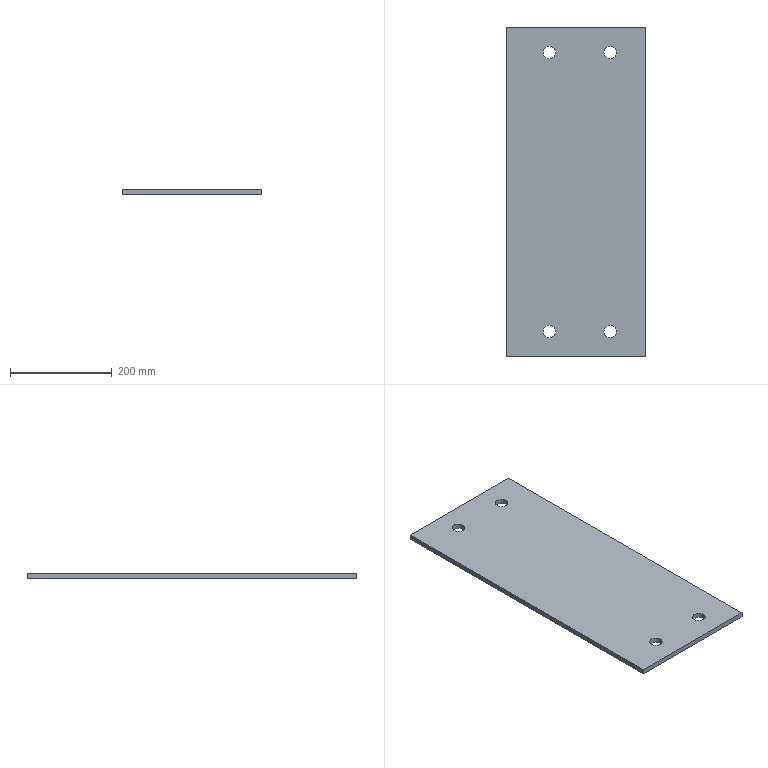Component | SolidWorks | Flange10-1 | 1 solid | 14 faces | box 275 x 650 x 10 mm | volume 1767865 mm3 | cylinder 8 | plane 6 | commonest cylinder face diameters 25 x8 | material Plain Carbon Steel
STEP:
#1=COLOUR_RGB('',0.7922,0.8196,0.9333);
#2=FILL_AREA_STYLE_COLOUR('',#1);
#3=FILL_AREA_STYLE('',(#2));
#4=SURFACE_STYLE_FILL_AREA(#3);
#5=SURFACE_SIDE_STYLE('',(#4));
#6=SURFACE_STYLE_USAGE(.BOTH.,#5);
#7=PRESENTATION_STYLE_ASSIGNMENT((#6));
#8=CARTESIAN_POINT('',(-129.713,64.816,204.172));
#9=VERTEX_POINT('',#8);
#10=CARTESIAN_POINT('',(-130.697,64.816,204.172));
#11=VERTEX_POINT('',#10);
#12=CARTESIAN_POINT('',(-130.205,64.816,204.172));
#13=DIRECTION('',(-0.,-0.,1.));
#14=DIRECTION('',(-1.,-0.,0.));
#15=AXIS2_PLACEMENT_3D('',#12,#13,#14);
#16=CIRCLE('',#15,0.4921);
#17=EDGE_CURVE('',#9,#11,#16,.T.);
#18=ORIENTED_EDGE('',*,*,#17,.F.);
#19=CARTESIAN_POINT('',(-129.713,64.816,204.566));
#20=VERTEX_POINT('',#19);
#21=CARTESIAN_POINT('',(-129.713,64.816,188.03));
#22=DIRECTION('',(-0.,-0.,1.));
#23=VECTOR('',#22,39.37);
#24=LINE('',#21,#23);
#25=EDGE_CURVE('',#9,#20,#24,.T.);
#26=ORIENTED_EDGE('',*,*,#25,.T.);
#27=CARTESIAN_POINT('',(-130.697,64.816,204.566));
#28=VERTEX_POINT('',#27);
#29=CARTESIAN_POINT('',(-130.205,64.816,204.566));
#30=DIRECTION('',(-0.,-0.,1.));
#31=DIRECTION('',(-1.,-0.,0.));
#32=AXIS2_PLACEMENT_3D('',#29,#30,#31);
#33=CIRCLE('',#32,0.4921);
#34=EDGE_CURVE('',#20,#28,#33,.T.);
#35=ORIENTED_EDGE('',*,*,#34,.T.);
#36=CARTESIAN_POINT('',(-130.697,64.816,188.03));
#37=DIRECTION('',(-0.,-0.,1.));
#38=VECTOR('',#37,39.37);
#39=LINE('',#36,#38);
#40=EDGE_CURVE('',#11,#28,#39,.T.);
#41=ORIENTED_EDGE('',*,*,#40,.F.);
#42=EDGE_LOOP('',(#18,#26,#35,#41));
#43=FACE_OUTER_BOUND('',#42,.T.);
#44=CARTESIAN_POINT('',(-130.205,64.816,188.03));
#45=DIRECTION('',(-0.,-0.,1.));
#46=DIRECTION('',(-1.,-0.,0.));
#47=AXIS2_PLACEMENT_3D('',#44,#45,#46);
#48=CYLINDRICAL_SURFACE('',#47,0.4921);
#49=ADVANCED_FACE('',(#43),#48,.F.);
#50=CARTESIAN_POINT('',(-124.988,86.469,204.172));
#51=VERTEX_POINT('',#50);
#52=CARTESIAN_POINT('',(-125.972,86.469,204.172));
#53=VERTEX_POINT('',#52);
#54=CARTESIAN_POINT('',(-125.48,86.469,204.172));
#55=DIRECTION('',(-0.,-0.,1.));
#56=DIRECTION('',(-1.,0.,0.));
#57=AXIS2_PLACEMENT_3D('',#54,#55,#56);
#58=CIRCLE('',#57,0.4921);
#59=EDGE_CURVE('',#51,#53,#58,.T.);
#60=ORIENTED_EDGE('',*,*,#59,.F.);
#61=CARTESIAN_POINT('',(-124.988,86.469,204.566));
#62=VERTEX_POINT('',#61);
#63=CARTESIAN_POINT('',(-124.988,86.469,188.03));
#64=DIRECTION('',(-0.,-0.,1.));
#65=VECTOR('',#64,39.37);
#66=LINE('',#63,#65);
#67=EDGE_CURVE('',#51,#62,#66,.T.);
#68=ORIENTED_EDGE('',*,*,#67,.T.);
#69=CARTESIAN_POINT('',(-125.972,86.469,204.566));
#70=VERTEX_POINT('',#69);
#71=CARTESIAN_POINT('',(-125.48,86.469,204.566));
#72=DIRECTION('',(-0.,-0.,1.));
#73=DIRECTION('',(-1.,0.,0.));
#74=AXIS2_PLACEMENT_3D('',#71,#72,#73);
#75=CIRCLE('',#74,0.4921);
#76=EDGE_CURVE('',#62,#70,#75,.T.);
#77=ORIENTED_EDGE('',*,*,#76,.T.);
#78=CARTESIAN_POINT('',(-125.972,86.469,188.03));
#79=DIRECTION('',(-0.,-0.,1.));
#80=VECTOR('',#79,39.37);
#81=LINE('',#78,#80);
#82=EDGE_CURVE('',#53,#70,#81,.T.);
#83=ORIENTED_EDGE('',*,*,#82,.F.);
#84=EDGE_LOOP('',(#60,#68,#77,#83));
#85=FACE_OUTER_BOUND('',#84,.T.);
#86=CARTESIAN_POINT('',(-125.48,86.469,188.03));
#87=DIRECTION('',(-0.,-0.,1.));
#88=DIRECTION('',(-1.,0.,0.));
#89=AXIS2_PLACEMENT_3D('',#86,#87,#88);
#90=CYLINDRICAL_SURFACE('',#89,0.4921);
#91=ADVANCED_FACE('',(#85),#90,.F.);
#92=CARTESIAN_POINT('',(-124.988,64.816,204.172));
#93=VERTEX_POINT('',#92);
#94=CARTESIAN_POINT('',(-125.972,64.816,204.172));
#95=VERTEX_POINT('',#94);
#96=CARTESIAN_POINT('',(-125.48,64.816,204.172));
#97=DIRECTION('',(-0.,-0.,1.));
#98=DIRECTION('',(-1.,-0.,0.));
#99=AXIS2_PLACEMENT_3D('',#96,#97,#98);
#100=CIRCLE('',#99,0.4921);
#101=EDGE_CURVE('',#93,#95,#100,.T.);
#102=ORIENTED_EDGE('',*,*,#101,.F.);
#103=CARTESIAN_POINT('',(-124.988,64.816,204.566));
#104=VERTEX_POINT('',#103);
#105=CARTESIAN_POINT('',(-124.988,64.816,188.03));
#106=DIRECTION('',(-0.,-0.,1.));
#107=VECTOR('',#106,39.37);
#108=LINE('',#105,#107);
#109=EDGE_CURVE('',#93,#104,#108,.T.);
#110=ORIENTED_EDGE('',*,*,#109,.T.);
#111=CARTESIAN_POINT('',(-125.972,64.816,204.566));
#112=VERTEX_POINT('',#111);
#113=CARTESIAN_POINT('',(-125.48,64.816,204.566));
#114=DIRECTION('',(-0.,-0.,1.));
#115=DIRECTION('',(-1.,-0.,0.));
#116=AXIS2_PLACEMENT_3D('',#113,#114,#115);
#117=CIRCLE('',#116,0.4921);
#118=EDGE_CURVE('',#104,#112,#117,.T.);
#119=ORIENTED_EDGE('',*,*,#118,.T.);
#120=CARTESIAN_POINT('',(-125.972,64.816,188.03));
#121=DIRECTION('',(-0.,-0.,1.));
#122=VECTOR('',#121,39.37);
#123=LINE('',#120,#122);
#124=EDGE_CURVE('',#95,#112,#123,.T.);
#125=ORIENTED_EDGE('',*,*,#124,.F.);
#126=EDGE_LOOP('',(#102,#110,#119,#125));
#127=FACE_OUTER_BOUND('',#126,.T.);
#128=CARTESIAN_POINT('',(-125.48,64.816,188.03));
#129=DIRECTION('',(-0.,-0.,1.));
#130=DIRECTION('',(-1.,-0.,0.));
#131=AXIS2_PLACEMENT_3D('',#128,#129,#130);
#132=CYLINDRICAL_SURFACE('',#131,0.4921);
#133=ADVANCED_FACE('',(#127),#132,.F.);
#134=CARTESIAN_POINT('',(-129.713,86.469,204.172));
#135=VERTEX_POINT('',#134);
#136=CARTESIAN_POINT('',(-130.697,86.469,204.172));
#137=VERTEX_POINT('',#136);
#138=CARTESIAN_POINT('',(-130.205,86.469,204.172));
#139=DIRECTION('',(-0.,-0.,1.));
#140=DIRECTION('',(-1.,0.,0.));
#141=AXIS2_PLACEMENT_3D('',#138,#139,#140);
#142=CIRCLE('',#141,0.4921);
#143=EDGE_CURVE('',#135,#137,#142,.T.);
#144=ORIENTED_EDGE('',*,*,#143,.F.);
#145=CARTESIAN_POINT('',(-129.713,86.469,204.566));
#146=VERTEX_POINT('',#145);
#147=CARTESIAN_POINT('',(-129.713,86.469,188.03));
#148=DIRECTION('',(-0.,-0.,1.));
#149=VECTOR('',#148,39.37);
#150=LINE('',#147,#149);
#151=EDGE_CURVE('',#135,#146,#150,.T.);
#152=ORIENTED_EDGE('',*,*,#151,.T.);
#153=CARTESIAN_POINT('',(-130.697,86.469,204.566));
#154=VERTEX_POINT('',#153);
#155=CARTESIAN_POINT('',(-130.205,86.469,204.566));
#156=DIRECTION('',(-0.,-0.,1.));
#157=DIRECTION('',(-1.,0.,0.));
#158=AXIS2_PLACEMENT_3D('',#155,#156,#157);
#159=CIRCLE('',#158,0.4921);
#160=EDGE_CURVE('',#146,#154,#159,.T.);
#161=ORIENTED_EDGE('',*,*,#160,.T.);
#162=CARTESIAN_POINT('',(-130.697,86.469,188.03));
#163=DIRECTION('',(-0.,-0.,1.));
#164=VECTOR('',#163,39.37);
#165=LINE('',#162,#164);
#166=EDGE_CURVE('',#137,#154,#165,.T.);
#167=ORIENTED_EDGE('',*,*,#166,.F.);
#168=EDGE_LOOP('',(#144,#152,#161,#167));
#169=FACE_OUTER_BOUND('',#168,.T.);
#170=CARTESIAN_POINT('',(-130.205,86.469,188.03));
#171=DIRECTION('',(-0.,-0.,1.));
#172=DIRECTION('',(-1.,0.,0.));
#173=AXIS2_PLACEMENT_3D('',#170,#171,#172);
#174=CYLINDRICAL_SURFACE('',#173,0.4921);
#175=ADVANCED_FACE('',(#169),#174,.F.);
#176=CARTESIAN_POINT('',(-133.551,88.438,204.566));
#177=VERTEX_POINT('',#176);
#178=CARTESIAN_POINT('',(-122.724,88.438,204.566));
#179=VERTEX_POINT('',#178);
#180=CARTESIAN_POINT('',(-133.551,88.438,204.566));
#181=DIRECTION('',(1.,0.,0.));
#182=VECTOR('',#181,39.37);
#183=LINE('',#180,#182);
#184=EDGE_CURVE('',#177,#179,#183,.T.);
#185=ORIENTED_EDGE('',*,*,#184,.T.);
#186=CARTESIAN_POINT('',(-122.724,88.438,204.172));
#187=VERTEX_POINT('',#186);
#188=CARTESIAN_POINT('',(-122.724,88.438,204.566));
#189=DIRECTION('',(0.,0.,-1.));
#190=VECTOR('',#189,39.37);
#191=LINE('',#188,#190);
#192=EDGE_CURVE('',#179,#187,#191,.T.);
#193=ORIENTED_EDGE('',*,*,#192,.T.);
#194=CARTESIAN_POINT('',(-133.551,88.438,204.172));
#195=VERTEX_POINT('',#194);
#196=CARTESIAN_POINT('',(-133.551,88.438,204.172));
#197=DIRECTION('',(1.,0.,0.));
#198=VECTOR('',#197,39.37);
#199=LINE('',#196,#198);
#200=EDGE_CURVE('',#195,#187,#199,.T.);
#201=ORIENTED_EDGE('',*,*,#200,.F.);
#202=CARTESIAN_POINT('',(-133.551,88.438,204.172));
#203=DIRECTION('',(-0.,-0.,1.));
#204=VECTOR('',#203,39.37);
#205=LINE('',#202,#204);
#206=EDGE_CURVE('',#195,#177,#205,.T.);
#207=ORIENTED_EDGE('',*,*,#206,.T.);
#208=EDGE_LOOP('',(#185,#193,#201,#207));
#209=FACE_OUTER_BOUND('',#208,.T.);
#210=CARTESIAN_POINT('',(-121.74,88.438,203.188));
#211=DIRECTION('',(-0.,1.,0.));
#212=DIRECTION('',(-1.,-0.,-0.));
#213=AXIS2_PLACEMENT_3D('',#210,#211,#212);
#214=PLANE('',#213);
#215=ADVANCED_FACE('',(#209),#214,.T.);
#216=CARTESIAN_POINT('',(-130.205,64.816,204.566));
#217=DIRECTION('',(-0.,-0.,1.));
#218=DIRECTION('',(-1.,-0.,0.));
#219=AXIS2_PLACEMENT_3D('',#216,#217,#218);
#220=CIRCLE('',#219,0.4921);
#221=EDGE_CURVE('',#28,#20,#220,.T.);
#222=ORIENTED_EDGE('',*,*,#221,.F.);
#223=ORIENTED_EDGE('',*,*,#34,.F.);
#224=EDGE_LOOP('',(#222,#223));
#225=FACE_BOUND('',#224,.T.);
#226=CARTESIAN_POINT('',(-125.48,86.469,204.566));
#227=DIRECTION('',(-0.,-0.,1.));
#228=DIRECTION('',(-1.,0.,0.));
#229=AXIS2_PLACEMENT_3D('',#226,#227,#228);
#230=CIRCLE('',#229,0.4921);
#231=EDGE_CURVE('',#70,#62,#230,.T.);
#232=ORIENTED_EDGE('',*,*,#231,.F.);
#233=ORIENTED_EDGE('',*,*,#76,.F.);
#234=EDGE_LOOP('',(#232,#233));
#235=FACE_BOUND('',#234,.T.);
#236=CARTESIAN_POINT('',(-125.48,64.816,204.566));
#237=DIRECTION('',(-0.,-0.,1.));
#238=DIRECTION('',(-1.,-0.,0.));
#239=AXIS2_PLACEMENT_3D('',#236,#237,#238);
#240=CIRCLE('',#239,0.4921);
#241=EDGE_CURVE('',#112,#104,#240,.T.);
#242=ORIENTED_EDGE('',*,*,#241,.F.);
#243=ORIENTED_EDGE('',*,*,#118,.F.);
#244=EDGE_LOOP('',(#242,#243));
#245=FACE_BOUND('',#244,.T.);
#246=CARTESIAN_POINT('',(-130.205,86.469,204.566));
#247=DIRECTION('',(-0.,-0.,1.));
#248=DIRECTION('',(-1.,0.,0.));
#249=AXIS2_PLACEMENT_3D('',#246,#247,#248);
#250=CIRCLE('',#249,0.4921);
#251=EDGE_CURVE('',#154,#146,#250,.T.);
#252=ORIENTED_EDGE('',*,*,#251,.F.);
#253=ORIENTED_EDGE('',*,*,#160,.F.);
#254=EDGE_LOOP('',(#252,#253));
#255=FACE_BOUND('',#254,.T.);
#256=ORIENTED_EDGE('',*,*,#184,.F.);
#257=CARTESIAN_POINT('',(-133.551,62.847,204.566));
#258=VERTEX_POINT('',#257);
#259=CARTESIAN_POINT('',(-133.551,62.847,204.566));
#260=DIRECTION('',(-0.,1.,0.));
#261=VECTOR('',#260,39.37);
#262=LINE('',#259,#261);
#263=EDGE_CURVE('',#258,#177,#262,.T.);
#264=ORIENTED_EDGE('',*,*,#263,.F.);
#265=CARTESIAN_POINT('',(-122.724,62.847,204.566));
#266=VERTEX_POINT('',#265);
#267=CARTESIAN_POINT('',(-133.551,62.847,204.566));
#268=DIRECTION('',(1.,0.,0.));
#269=VECTOR('',#268,39.37);
#270=LINE('',#267,#269);
#271=EDGE_CURVE('',#258,#266,#270,.T.);
#272=ORIENTED_EDGE('',*,*,#271,.T.);
#273=CARTESIAN_POINT('',(-122.724,62.847,204.566));
#274=DIRECTION('',(-0.,1.,0.));
#275=VECTOR('',#274,39.37);
#276=LINE('',#273,#275);
#277=EDGE_CURVE('',#266,#179,#276,.T.);
#278=ORIENTED_EDGE('',*,*,#277,.T.);
#279=EDGE_LOOP('',(#256,#264,#272,#278));
#280=FACE_OUTER_BOUND('',#279,.T.);
#281=CARTESIAN_POINT('',(-133.551,62.847,204.566));
#282=DIRECTION('',(-0.,-0.,1.));
#283=DIRECTION('',(-1.,-0.,-0.));
#284=AXIS2_PLACEMENT_3D('',#281,#282,#283);
#285=PLANE('',#284);
#286=ADVANCED_FACE('',(#225,#235,#245,#255,#280),#285,.T.);
#287=ORIENTED_EDGE('',*,*,#206,.F.);
#288=CARTESIAN_POINT('',(-133.551,62.847,204.172));
#289=VERTEX_POINT('',#288);
#290=CARTESIAN_POINT('',(-133.551,62.847,204.172));
#291=DIRECTION('',(-0.,1.,0.));
#292=VECTOR('',#291,39.37);
#293=LINE('',#290,#292);
#294=EDGE_CURVE('',#289,#195,#293,.T.);
#295=ORIENTED_EDGE('',*,*,#294,.F.);
#296=CARTESIAN_POINT('',(-133.551,62.847,204.172));
#297=DIRECTION('',(-0.,-0.,1.));
#298=VECTOR('',#297,39.37);
#299=LINE('',#296,#298);
#300=EDGE_CURVE('',#289,#258,#299,.T.);
#301=ORIENTED_EDGE('',*,*,#300,.T.);
#302=ORIENTED_EDGE('',*,*,#263,.T.);
#303=EDGE_LOOP('',(#287,#295,#301,#302));
#304=FACE_OUTER_BOUND('',#303,.T.);
#305=CARTESIAN_POINT('',(-133.551,62.847,204.172));
#306=DIRECTION('',(-1.,-0.,-0.));
#307=DIRECTION('',(0.,-1.,-0.));
#308=AXIS2_PLACEMENT_3D('',#305,#306,#307);
#309=PLANE('',#308);
#310=ADVANCED_FACE('',(#304),#309,.T.);
#311=CARTESIAN_POINT('',(-130.205,64.816,204.172));
#312=DIRECTION('',(-0.,-0.,1.));
#313=DIRECTION('',(-1.,-0.,0.));
#314=AXIS2_PLACEMENT_3D('',#311,#312,#313);
#315=CIRCLE('',#314,0.4921);
#316=EDGE_CURVE('',#11,#9,#315,.T.);
#317=ORIENTED_EDGE('',*,*,#316,.T.);
#318=ORIENTED_EDGE('',*,*,#17,.T.);
#319=EDGE_LOOP('',(#317,#318));
#320=FACE_BOUND('',#319,.T.);
#321=CARTESIAN_POINT('',(-125.48,86.469,204.172));
#322=DIRECTION('',(-0.,-0.,1.));
#323=DIRECTION('',(-1.,0.,0.));
#324=AXIS2_PLACEMENT_3D('',#321,#322,#323);
#325=CIRCLE('',#324,0.4921);
#326=EDGE_CURVE('',#53,#51,#325,.T.);
#327=ORIENTED_EDGE('',*,*,#326,.T.);
#328=ORIENTED_EDGE('',*,*,#59,.T.);
#329=EDGE_LOOP('',(#327,#328));
#330=FACE_BOUND('',#329,.T.);
#331=CARTESIAN_POINT('',(-125.48,64.816,204.172));
#332=DIRECTION('',(-0.,-0.,1.));
#333=DIRECTION('',(-1.,-0.,0.));
#334=AXIS2_PLACEMENT_3D('',#331,#332,#333);
#335=CIRCLE('',#334,0.4921);
#336=EDGE_CURVE('',#95,#93,#335,.T.);
#337=ORIENTED_EDGE('',*,*,#336,.T.);
#338=ORIENTED_EDGE('',*,*,#101,.T.);
#339=EDGE_LOOP('',(#337,#338));
#340=FACE_BOUND('',#339,.T.);
#341=CARTESIAN_POINT('',(-130.205,86.469,204.172));
#342=DIRECTION('',(-0.,-0.,1.));
#343=DIRECTION('',(-1.,0.,0.));
#344=AXIS2_PLACEMENT_3D('',#341,#342,#343);
#345=CIRCLE('',#344,0.4921);
#346=EDGE_CURVE('',#137,#135,#345,.T.);
#347=ORIENTED_EDGE('',*,*,#346,.T.);
#348=ORIENTED_EDGE('',*,*,#143,.T.);
#349=EDGE_LOOP('',(#347,#348));
#350=FACE_BOUND('',#349,.T.);
#351=ORIENTED_EDGE('',*,*,#200,.T.);
#352=CARTESIAN_POINT('',(-122.724,62.847,204.172));
#353=VERTEX_POINT('',#352);
#354=CARTESIAN_POINT('',(-122.724,62.847,204.172));
#355=DIRECTION('',(-0.,1.,0.));
#356=VECTOR('',#355,39.37);
#357=LINE('',#354,#356);
#358=EDGE_CURVE('',#353,#187,#357,.T.);
#359=ORIENTED_EDGE('',*,*,#358,.F.);
#360=CARTESIAN_POINT('',(-133.551,62.847,204.172));
#361=DIRECTION('',(1.,0.,0.));
#362=VECTOR('',#361,39.37);
#363=LINE('',#360,#362);
#364=EDGE_CURVE('',#289,#353,#363,.T.);
#365=ORIENTED_EDGE('',*,*,#364,.F.);
#366=ORIENTED_EDGE('',*,*,#294,.T.);
#367=EDGE_LOOP('',(#351,#359,#365,#366));
#368=FACE_OUTER_BOUND('',#367,.T.);
#369=CARTESIAN_POINT('',(-133.551,62.847,204.172));
#370=DIRECTION('',(-0.,-0.,1.));
#371=DIRECTION('',(-1.,-0.,-0.));
#372=AXIS2_PLACEMENT_3D('',#369,#370,#371);
#373=PLANE('',#372);
#374=ADVANCED_FACE('',(#320,#330,#340,#350,#368),#373,.F.);
#375=ORIENTED_EDGE('',*,*,#364,.T.);
#376=CARTESIAN_POINT('',(-122.724,62.847,204.172));
#377=DIRECTION('',(-0.,-0.,1.));
#378=VECTOR('',#377,39.37);
#379=LINE('',#376,#378);
#380=EDGE_CURVE('',#353,#266,#379,.T.);
#381=ORIENTED_EDGE('',*,*,#380,.T.);
#382=ORIENTED_EDGE('',*,*,#271,.F.);
#383=ORIENTED_EDGE('',*,*,#300,.F.);
#384=EDGE_LOOP('',(#375,#381,#382,#383));
#385=FACE_OUTER_BOUND('',#384,.T.);
#386=CARTESIAN_POINT('',(-122.724,62.847,203.188));
#387=DIRECTION('',(0.,-1.,-0.));
#388=DIRECTION('',(1.,0.,0.));
#389=AXIS2_PLACEMENT_3D('',#386,#387,#388);
#390=PLANE('',#389);
#391=ADVANCED_FACE('',(#385),#390,.T.);
#392=ORIENTED_EDGE('',*,*,#151,.F.);
#393=ORIENTED_EDGE('',*,*,#346,.F.);
#394=ORIENTED_EDGE('',*,*,#166,.T.);
#395=ORIENTED_EDGE('',*,*,#251,.T.);
#396=EDGE_LOOP('',(#392,#393,#394,#395));
#397=FACE_OUTER_BOUND('',#396,.T.);
#398=CARTESIAN_POINT('',(-130.205,86.469,188.03));
#399=DIRECTION('',(-0.,-0.,1.));
#400=DIRECTION('',(-1.,0.,0.));
#401=AXIS2_PLACEMENT_3D('',#398,#399,#400);
#402=CYLINDRICAL_SURFACE('',#401,0.4921);
#403=ADVANCED_FACE('',(#397),#402,.F.);
#404=ORIENTED_EDGE('',*,*,#109,.F.);
#405=ORIENTED_EDGE('',*,*,#336,.F.);
#406=ORIENTED_EDGE('',*,*,#124,.T.);
#407=ORIENTED_EDGE('',*,*,#241,.T.);
#408=EDGE_LOOP('',(#404,#405,#406,#407));
#409=FACE_OUTER_BOUND('',#408,.T.);
#410=CARTESIAN_POINT('',(-125.48,64.816,188.03));
#411=DIRECTION('',(-0.,-0.,1.));
#412=DIRECTION('',(-1.,-0.,0.));
#413=AXIS2_PLACEMENT_3D('',#410,#411,#412);
#414=CYLINDRICAL_SURFACE('',#413,0.4921);
#415=ADVANCED_FACE('',(#409),#414,.F.);
#416=ORIENTED_EDGE('',*,*,#67,.F.);
#417=ORIENTED_EDGE('',*,*,#326,.F.);
#418=ORIENTED_EDGE('',*,*,#82,.T.);
#419=ORIENTED_EDGE('',*,*,#231,.T.);
#420=EDGE_LOOP('',(#416,#417,#418,#419));
#421=FACE_OUTER_BOUND('',#420,.T.);
#422=CARTESIAN_POINT('',(-125.48,86.469,188.03));
#423=DIRECTION('',(-0.,-0.,1.));
#424=DIRECTION('',(-1.,0.,0.));
#425=AXIS2_PLACEMENT_3D('',#422,#423,#424);
#426=CYLINDRICAL_SURFACE('',#425,0.4921);
#427=ADVANCED_FACE('',(#421),#426,.F.);
#428=ORIENTED_EDGE('',*,*,#25,.F.);
#429=ORIENTED_EDGE('',*,*,#316,.F.);
#430=ORIENTED_EDGE('',*,*,#40,.T.);
#431=ORIENTED_EDGE('',*,*,#221,.T.);
#432=EDGE_LOOP('',(#428,#429,#430,#431));
#433=FACE_OUTER_BOUND('',#432,.T.);
#434=CARTESIAN_POINT('',(-130.205,64.816,188.03));
#435=DIRECTION('',(-0.,-0.,1.));
#436=DIRECTION('',(-1.,-0.,0.));
#437=AXIS2_PLACEMENT_3D('',#434,#435,#436);
#438=CYLINDRICAL_SURFACE('',#437,0.4921);
#439=ADVANCED_FACE('',(#433),#438,.F.);
#440=ORIENTED_EDGE('',*,*,#192,.F.);
#441=ORIENTED_EDGE('',*,*,#277,.F.);
#442=ORIENTED_EDGE('',*,*,#380,.F.);
#443=ORIENTED_EDGE('',*,*,#358,.T.);
#444=EDGE_LOOP('',(#440,#441,#442,#443));
#445=FACE_OUTER_BOUND('',#444,.T.);
#446=CARTESIAN_POINT('',(-122.724,88.438,188.03));
#447=DIRECTION('',(-1.,-0.,-0.));
#448=DIRECTION('',(0.,-1.,-0.));
#449=AXIS2_PLACEMENT_3D('',#446,#447,#448);
#450=PLANE('',#449);
#451=ADVANCED_FACE('',(#445),#450,.F.);
#452=CLOSED_SHELL('',(#49,#91,#133,#175,#215,#286,#310,#374,#391,#403,#415,#427,#439,#451));
#453=MANIFOLD_SOLID_BREP('',#452);
#454=STYLED_ITEM('',(#7),#453);
#455=(LENGTH_UNIT()NAMED_UNIT(*)SI_UNIT($,.METRE.));
#456=LENGTH_MEASURE_WITH_UNIT(LENGTH_MEASURE(0.0254),#455);
#457=DIMENSIONAL_EXPONENTS(1.,0.,0.,0.,0.,0.,0.);
#458=(CONVERSION_BASED_UNIT('',#456)LENGTH_UNIT()NAMED_UNIT(#457));
#459=UNCERTAINTY_MEASURE_WITH_UNIT(LENGTH_MEASURE(0.00001),#458,'','');
#460=(NAMED_UNIT(*)PLANE_ANGLE_UNIT()SI_UNIT($,.RADIAN.));
#461=(NAMED_UNIT(*)SI_UNIT($,.STERADIAN.)SOLID_ANGLE_UNIT());
#462=(GEOMETRIC_REPRESENTATION_CONTEXT(3)GLOBAL_UNCERTAINTY_ASSIGNED_CONTEXT((#459))GLOBAL_UNIT_ASSIGNED_CONTEXT((#458,#460,#461))REPRESENTATION_CONTEXT('',''));
#463=MECHANICAL_DESIGN_GEOMETRIC_PRESENTATION_REPRESENTATION('',(#454),#462);
#464=PRESENTATION_LAYER_ASSIGNMENT('','',(#454));
#465=CARTESIAN_POINT('',(0.,0.,0.));
#466=DIRECTION('',(0.,0.,1.));
#467=DIRECTION('',(1.,0.,0.));
#468=AXIS2_PLACEMENT_3D('',#465,#466,#467);
#469=(LENGTH_UNIT()NAMED_UNIT(*)SI_UNIT($,.METRE.));
#470=LENGTH_MEASURE_WITH_UNIT(LENGTH_MEASURE(0.0254),#469);
#471=DIMENSIONAL_EXPONENTS(1.,0.,0.,0.,0.,0.,0.);
#472=(CONVERSION_BASED_UNIT('',#470)LENGTH_UNIT()NAMED_UNIT(#471));
#473=UNCERTAINTY_MEASURE_WITH_UNIT(LENGTH_MEASURE(0.00001),#472,'','');
#474=(NAMED_UNIT(*)PLANE_ANGLE_UNIT()SI_UNIT($,.RADIAN.));
#475=(NAMED_UNIT(*)SI_UNIT($,.STERADIAN.)SOLID_ANGLE_UNIT());
#476=(GEOMETRIC_REPRESENTATION_CONTEXT(3)GLOBAL_UNCERTAINTY_ASSIGNED_CONTEXT((#473))GLOBAL_UNIT_ASSIGNED_CONTEXT((#472,#474,#475))REPRESENTATION_CONTEXT('',''));
#477=ADVANCED_BREP_SHAPE_REPRESENTATION('',(#453,#468),#476);